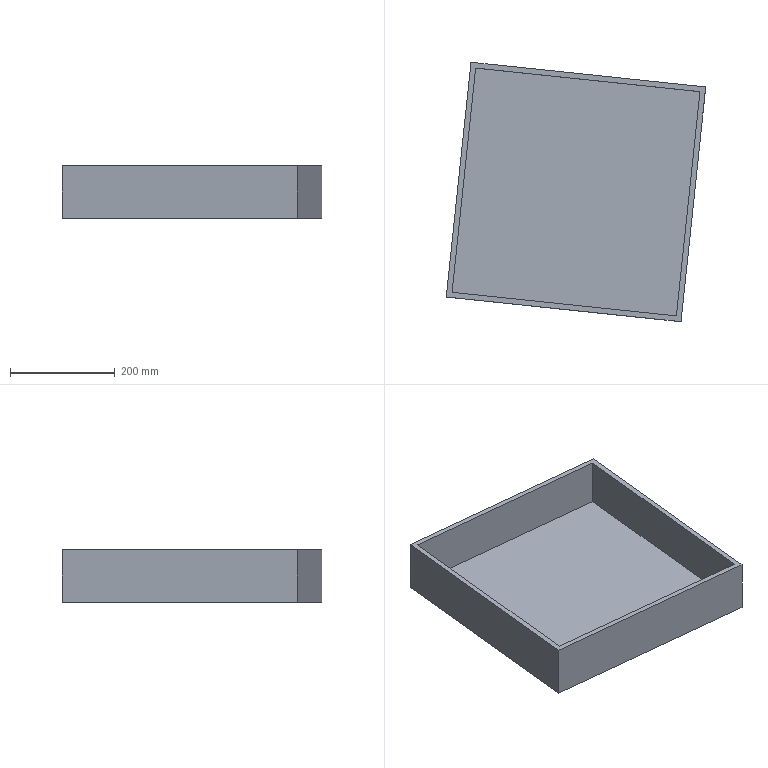Component | NX | STORAGE_BOX | 1 solid | 11 faces | box 494.57 x 494.57 x 100 mm | volume 3609000 mm3 | plane 11
STEP:
#1=CARTESIAN_POINT('',(0.,0.,0.));
#2=DIRECTION('',(0.,0.,1.));
#3=DIRECTION('',(1.,0.,0.));
#4=AXIS2_PLACEMENT_3D('',#1,#2,#3);
#5=CARTESIAN_POINT('',(1089.335,1116.284,120.));
#6=VERTEX_POINT('',#5);
#7=CARTESIAN_POINT('',(1042.297,668.75,120.));
#8=VERTEX_POINT('',#7);
#9=CARTESIAN_POINT('',(1065.816,892.517,120.));
#10=DIRECTION('',(-0.1045,-0.9945,0.));
#11=VECTOR('',#10,1.);
#12=LINE('',#9,#11);
#13=CARTESIAN_POINT('',(842.048,916.036,120.));
#14=DIRECTION('',(0.,0.,1.));
#15=DIRECTION('',(0.1045,0.9945,0.));
#16=AXIS2_PLACEMENT_3D('',#13,#14,#15);
#17=PLANE('',#16);
#18=CARTESIAN_POINT('',(-0.,-225.));
#19=DIRECTION('',(-1.,0.));
#20=VECTOR('',#19,1.);
#21=LINE('',#18,#20);
#22=(GEOMETRIC_REPRESENTATION_CONTEXT(2)PARAMETRIC_REPRESENTATION_CONTEXT()REPRESENTATION_CONTEXT('',''));
#23=DEFINITIONAL_REPRESENTATION('',(#21),#22);
#24=PCURVE('',#17,#23);
#25=CARTESIAN_POINT('',(1065.816,892.517,20.));
#26=DIRECTION('',(0.9945,-0.1045,0.));
#27=DIRECTION('',(0.,0.,-1.));
#28=AXIS2_PLACEMENT_3D('',#25,#26,#27);
#29=PLANE('',#28);
#30=CARTESIAN_POINT('',(-100.,0.));
#31=DIRECTION('',(0.,-1.));
#32=VECTOR('',#31,1.);
#33=LINE('',#30,#32);
#34=(GEOMETRIC_REPRESENTATION_CONTEXT(2)PARAMETRIC_REPRESENTATION_CONTEXT()REPRESENTATION_CONTEXT('',''));
#35=DEFINITIONAL_REPRESENTATION('',(#33),#34);
#36=PCURVE('',#29,#35);
#37=SURFACE_CURVE('',#12,(#24,#36),.PCURVE_S1.);
#38=EDGE_CURVE('',#6,#8,#37,.T.);
#39=ORIENTED_EDGE('',*,*,#38,.F.);
#40=CARTESIAN_POINT('',(641.8,1163.322,120.));
#41=VERTEX_POINT('',#40);
#42=CARTESIAN_POINT('',(865.567,1139.803,120.));
#43=DIRECTION('',(0.9945,-0.1045,0.));
#44=VECTOR('',#43,1.);
#45=LINE('',#42,#44);
#46=CARTESIAN_POINT('',(225.,-0.));
#47=DIRECTION('',(0.,-1.));
#48=VECTOR('',#47,1.);
#49=LINE('',#46,#48);
#50=(GEOMETRIC_REPRESENTATION_CONTEXT(2)PARAMETRIC_REPRESENTATION_CONTEXT()REPRESENTATION_CONTEXT('',''));
#51=DEFINITIONAL_REPRESENTATION('',(#49),#50);
#52=PCURVE('',#17,#51);
#53=CARTESIAN_POINT('',(865.567,1139.803,20.));
#54=DIRECTION('',(0.1045,0.9945,0.));
#55=DIRECTION('',(0.,0.,-1.));
#56=AXIS2_PLACEMENT_3D('',#53,#54,#55);
#57=PLANE('',#56);
#58=CARTESIAN_POINT('',(-100.,0.));
#59=DIRECTION('',(0.,-1.));
#60=VECTOR('',#59,1.);
#61=LINE('',#58,#60);
#62=(GEOMETRIC_REPRESENTATION_CONTEXT(2)PARAMETRIC_REPRESENTATION_CONTEXT()REPRESENTATION_CONTEXT('',''));
#63=DEFINITIONAL_REPRESENTATION('',(#61),#62);
#64=PCURVE('',#57,#63);
#65=SURFACE_CURVE('',#45,(#52,#64),.PCURVE_S1.);
#66=EDGE_CURVE('',#41,#6,#65,.T.);
#67=ORIENTED_EDGE('',*,*,#66,.F.);
#68=CARTESIAN_POINT('',(594.762,715.787,120.));
#69=VERTEX_POINT('',#68);
#70=CARTESIAN_POINT('',(618.281,939.555,120.));
#71=DIRECTION('',(0.1045,0.9945,0.));
#72=VECTOR('',#71,1.);
#73=LINE('',#70,#72);
#74=CARTESIAN_POINT('',(-0.,225.));
#75=DIRECTION('',(1.,0.));
#76=VECTOR('',#75,1.);
#77=LINE('',#74,#76);
#78=(GEOMETRIC_REPRESENTATION_CONTEXT(2)PARAMETRIC_REPRESENTATION_CONTEXT()REPRESENTATION_CONTEXT('',''));
#79=DEFINITIONAL_REPRESENTATION('',(#77),#78);
#80=PCURVE('',#17,#79);
#81=CARTESIAN_POINT('',(618.281,939.555,20.));
#82=DIRECTION('',(-0.9945,0.1045,0.));
#83=DIRECTION('',(0.,0.,1.));
#84=AXIS2_PLACEMENT_3D('',#81,#82,#83);
#85=PLANE('',#84);
#86=CARTESIAN_POINT('',(100.,0.));
#87=DIRECTION('',(0.,1.));
#88=VECTOR('',#87,1.);
#89=LINE('',#86,#88);
#90=(GEOMETRIC_REPRESENTATION_CONTEXT(2)PARAMETRIC_REPRESENTATION_CONTEXT()REPRESENTATION_CONTEXT('',''));
#91=DEFINITIONAL_REPRESENTATION('',(#89),#90);
#92=PCURVE('',#85,#91);
#93=SURFACE_CURVE('',#73,(#80,#92),.PCURVE_S1.);
#94=EDGE_CURVE('',#69,#41,#93,.T.);
#95=ORIENTED_EDGE('',*,*,#94,.F.);
#96=CARTESIAN_POINT('',(818.529,692.268,120.));
#97=DIRECTION('',(-0.9945,0.1045,0.));
#98=VECTOR('',#97,1.);
#99=LINE('',#96,#98);
#100=CARTESIAN_POINT('',(-225.,-0.));
#101=DIRECTION('',(0.,1.));
#102=VECTOR('',#101,1.);
#103=LINE('',#100,#102);
#104=(GEOMETRIC_REPRESENTATION_CONTEXT(2)PARAMETRIC_REPRESENTATION_CONTEXT()REPRESENTATION_CONTEXT('',''));
#105=DEFINITIONAL_REPRESENTATION('',(#103),#104);
#106=PCURVE('',#17,#105);
#107=CARTESIAN_POINT('',(818.529,692.268,20.));
#108=DIRECTION('',(-0.1045,-0.9945,0.));
#109=DIRECTION('',(0.,0.,1.));
#110=AXIS2_PLACEMENT_3D('',#107,#108,#109);
#111=PLANE('',#110);
#112=CARTESIAN_POINT('',(100.,0.));
#113=DIRECTION('',(0.,1.));
#114=VECTOR('',#113,1.);
#115=LINE('',#112,#114);
#116=(GEOMETRIC_REPRESENTATION_CONTEXT(2)PARAMETRIC_REPRESENTATION_CONTEXT()REPRESENTATION_CONTEXT('',''));
#117=DEFINITIONAL_REPRESENTATION('',(#115),#116);
#118=PCURVE('',#111,#117);
#119=SURFACE_CURVE('',#99,(#106,#118),.PCURVE_S1.);
#120=EDGE_CURVE('',#8,#69,#119,.T.);
#121=ORIENTED_EDGE('',*,*,#120,.F.);
#122=EDGE_LOOP('',(#39,#67,#95,#121));
#123=FACE_BOUND('',#122,.T.);
#124=CARTESIAN_POINT('',(650.7,1152.332,120.));
#125=VERTEX_POINT('',#124);
#126=CARTESIAN_POINT('',(1078.344,1107.384,120.));
#127=VERTEX_POINT('',#126);
#128=CARTESIAN_POINT('',(864.522,1129.858,120.));
#129=DIRECTION('',(0.9945,-0.1045,0.));
#130=VECTOR('',#129,1.);
#131=LINE('',#128,#130);
#132=CARTESIAN_POINT('',(215.,0.));
#133=DIRECTION('',(0.,-1.));
#134=VECTOR('',#133,1.);
#135=LINE('',#132,#134);
#136=(GEOMETRIC_REPRESENTATION_CONTEXT(2)PARAMETRIC_REPRESENTATION_CONTEXT()REPRESENTATION_CONTEXT('',''));
#137=DEFINITIONAL_REPRESENTATION('',(#135),#136);
#138=PCURVE('',#17,#137);
#139=CARTESIAN_POINT('',(864.522,1129.858,20.));
#140=DIRECTION('',(0.1045,0.9945,0.));
#141=DIRECTION('',(0.,0.,-1.));
#142=AXIS2_PLACEMENT_3D('',#139,#140,#141);
#143=PLANE('',#142);
#144=CARTESIAN_POINT('',(-100.,0.));
#145=DIRECTION('',(0.,-1.));
#146=VECTOR('',#145,1.);
#147=LINE('',#144,#146);
#148=(GEOMETRIC_REPRESENTATION_CONTEXT(2)PARAMETRIC_REPRESENTATION_CONTEXT()REPRESENTATION_CONTEXT('',''));
#149=DEFINITIONAL_REPRESENTATION('',(#147),#148);
#150=PCURVE('',#143,#149);
#151=SURFACE_CURVE('',#131,(#138,#150),.PCURVE_S1.);
#152=EDGE_CURVE('',#125,#127,#151,.T.);
#153=ORIENTED_EDGE('',*,*,#152,.T.);
#154=CARTESIAN_POINT('',(1033.397,679.74,120.));
#155=VERTEX_POINT('',#154);
#156=CARTESIAN_POINT('',(1055.871,893.562,120.));
#157=DIRECTION('',(-0.1045,-0.9945,0.));
#158=VECTOR('',#157,1.);
#159=LINE('',#156,#158);
#160=CARTESIAN_POINT('',(-0.,-215.));
#161=DIRECTION('',(-1.,0.));
#162=VECTOR('',#161,1.);
#163=LINE('',#160,#162);
#164=(GEOMETRIC_REPRESENTATION_CONTEXT(2)PARAMETRIC_REPRESENTATION_CONTEXT()REPRESENTATION_CONTEXT('',''));
#165=DEFINITIONAL_REPRESENTATION('',(#163),#164);
#166=PCURVE('',#17,#165);
#167=CARTESIAN_POINT('',(1055.871,893.562,20.));
#168=DIRECTION('',(0.9945,-0.1045,0.));
#169=DIRECTION('',(0.,0.,-1.));
#170=AXIS2_PLACEMENT_3D('',#167,#168,#169);
#171=PLANE('',#170);
#172=CARTESIAN_POINT('',(-100.,0.));
#173=DIRECTION('',(0.,-1.));
#174=VECTOR('',#173,1.);
#175=LINE('',#172,#174);
#176=(GEOMETRIC_REPRESENTATION_CONTEXT(2)PARAMETRIC_REPRESENTATION_CONTEXT()REPRESENTATION_CONTEXT('',''));
#177=DEFINITIONAL_REPRESENTATION('',(#175),#176);
#178=PCURVE('',#171,#177);
#179=SURFACE_CURVE('',#159,(#166,#178),.PCURVE_S1.);
#180=EDGE_CURVE('',#127,#155,#179,.T.);
#181=ORIENTED_EDGE('',*,*,#180,.T.);
#182=CARTESIAN_POINT('',(605.753,724.687,120.));
#183=VERTEX_POINT('',#182);
#184=CARTESIAN_POINT('',(819.575,702.214,120.));
#185=DIRECTION('',(-0.9945,0.1045,0.));
#186=VECTOR('',#185,1.);
#187=LINE('',#184,#186);
#188=CARTESIAN_POINT('',(-215.,0.));
#189=DIRECTION('',(0.,1.));
#190=VECTOR('',#189,1.);
#191=LINE('',#188,#190);
#192=(GEOMETRIC_REPRESENTATION_CONTEXT(2)PARAMETRIC_REPRESENTATION_CONTEXT()REPRESENTATION_CONTEXT('',''));
#193=DEFINITIONAL_REPRESENTATION('',(#191),#192);
#194=PCURVE('',#17,#193);
#195=CARTESIAN_POINT('',(819.575,702.214,20.));
#196=DIRECTION('',(-0.1045,-0.9945,0.));
#197=DIRECTION('',(0.,0.,1.));
#198=AXIS2_PLACEMENT_3D('',#195,#196,#197);
#199=PLANE('',#198);
#200=CARTESIAN_POINT('',(100.,0.));
#201=DIRECTION('',(0.,1.));
#202=VECTOR('',#201,1.);
#203=LINE('',#200,#202);
#204=(GEOMETRIC_REPRESENTATION_CONTEXT(2)PARAMETRIC_REPRESENTATION_CONTEXT()REPRESENTATION_CONTEXT('',''));
#205=DEFINITIONAL_REPRESENTATION('',(#203),#204);
#206=PCURVE('',#199,#205);
#207=SURFACE_CURVE('',#187,(#194,#206),.PCURVE_S1.);
#208=EDGE_CURVE('',#155,#183,#207,.T.);
#209=ORIENTED_EDGE('',*,*,#208,.T.);
#210=CARTESIAN_POINT('',(628.226,938.509,120.));
#211=DIRECTION('',(0.1045,0.9945,0.));
#212=VECTOR('',#211,1.);
#213=LINE('',#210,#212);
#214=CARTESIAN_POINT('',(-0.,215.));
#215=DIRECTION('',(1.,0.));
#216=VECTOR('',#215,1.);
#217=LINE('',#214,#216);
#218=(GEOMETRIC_REPRESENTATION_CONTEXT(2)PARAMETRIC_REPRESENTATION_CONTEXT()REPRESENTATION_CONTEXT('',''));
#219=DEFINITIONAL_REPRESENTATION('',(#217),#218);
#220=PCURVE('',#17,#219);
#221=CARTESIAN_POINT('',(628.226,938.509,20.));
#222=DIRECTION('',(-0.9945,0.1045,0.));
#223=DIRECTION('',(0.,0.,1.));
#224=AXIS2_PLACEMENT_3D('',#221,#222,#223);
#225=PLANE('',#224);
#226=CARTESIAN_POINT('',(100.,0.));
#227=DIRECTION('',(0.,1.));
#228=VECTOR('',#227,1.);
#229=LINE('',#226,#228);
#230=(GEOMETRIC_REPRESENTATION_CONTEXT(2)PARAMETRIC_REPRESENTATION_CONTEXT()REPRESENTATION_CONTEXT('',''));
#231=DEFINITIONAL_REPRESENTATION('',(#229),#230);
#232=PCURVE('',#225,#231);
#233=SURFACE_CURVE('',#213,(#220,#232),.PCURVE_S1.);
#234=EDGE_CURVE('',#183,#125,#233,.T.);
#235=ORIENTED_EDGE('',*,*,#234,.T.);
#236=EDGE_LOOP('',(#153,#181,#209,#235));
#237=FACE_BOUND('',#236,.T.);
#238=ADVANCED_FACE('',(#123,#237),#17,.T.);
#239=CARTESIAN_POINT('',(1089.335,1116.284,20.));
#240=VERTEX_POINT('',#239);
#241=CARTESIAN_POINT('',(1089.335,1116.284,20.));
#242=DIRECTION('',(0.,0.,1.));
#243=VECTOR('',#242,1.);
#244=LINE('',#241,#243);
#245=CARTESIAN_POINT('',(0.,225.));
#246=DIRECTION('',(-1.,0.));
#247=VECTOR('',#246,1.);
#248=LINE('',#245,#247);
#249=(GEOMETRIC_REPRESENTATION_CONTEXT(2)PARAMETRIC_REPRESENTATION_CONTEXT()REPRESENTATION_CONTEXT('',''));
#250=DEFINITIONAL_REPRESENTATION('',(#248),#249);
#251=PCURVE('',#29,#250);
#252=CARTESIAN_POINT('',(0.,-225.));
#253=DIRECTION('',(-1.,0.));
#254=VECTOR('',#253,1.);
#255=LINE('',#252,#254);
#256=(GEOMETRIC_REPRESENTATION_CONTEXT(2)PARAMETRIC_REPRESENTATION_CONTEXT()REPRESENTATION_CONTEXT('',''));
#257=DEFINITIONAL_REPRESENTATION('',(#255),#256);
#258=PCURVE('',#57,#257);
#259=SURFACE_CURVE('',#244,(#251,#258),.PCURVE_S1.);
#260=EDGE_CURVE('',#240,#6,#259,.T.);
#261=ORIENTED_EDGE('',*,*,#260,.T.);
#262=ORIENTED_EDGE('',*,*,#38,.T.);
#263=CARTESIAN_POINT('',(1042.297,668.75,20.));
#264=VERTEX_POINT('',#263);
#265=CARTESIAN_POINT('',(1042.297,668.75,20.));
#266=DIRECTION('',(0.,0.,1.));
#267=VECTOR('',#266,1.);
#268=LINE('',#265,#267);
#269=CARTESIAN_POINT('',(0.,-225.));
#270=DIRECTION('',(-1.,0.));
#271=VECTOR('',#270,1.);
#272=LINE('',#269,#271);
#273=(GEOMETRIC_REPRESENTATION_CONTEXT(2)PARAMETRIC_REPRESENTATION_CONTEXT()REPRESENTATION_CONTEXT('',''));
#274=DEFINITIONAL_REPRESENTATION('',(#272),#273);
#275=PCURVE('',#29,#274);
#276=CARTESIAN_POINT('',(0.,-225.));
#277=DIRECTION('',(1.,0.));
#278=VECTOR('',#277,1.);
#279=LINE('',#276,#278);
#280=(GEOMETRIC_REPRESENTATION_CONTEXT(2)PARAMETRIC_REPRESENTATION_CONTEXT()REPRESENTATION_CONTEXT('',''));
#281=DEFINITIONAL_REPRESENTATION('',(#279),#280);
#282=PCURVE('',#111,#281);
#283=SURFACE_CURVE('',#268,(#275,#282),.PCURVE_S1.);
#284=EDGE_CURVE('',#264,#8,#283,.T.);
#285=ORIENTED_EDGE('',*,*,#284,.F.);
#286=CARTESIAN_POINT('',(1065.816,892.517,20.));
#287=DIRECTION('',(0.1045,0.9945,0.));
#288=VECTOR('',#287,1.);
#289=LINE('',#286,#288);
#290=CARTESIAN_POINT('',(0.,0.));
#291=DIRECTION('',(0.,1.));
#292=VECTOR('',#291,1.);
#293=LINE('',#290,#292);
#294=(GEOMETRIC_REPRESENTATION_CONTEXT(2)PARAMETRIC_REPRESENTATION_CONTEXT()REPRESENTATION_CONTEXT('',''));
#295=DEFINITIONAL_REPRESENTATION('',(#293),#294);
#296=PCURVE('',#29,#295);
#297=CARTESIAN_POINT('',(842.048,916.036,20.));
#298=DIRECTION('',(0.,0.,-1.));
#299=DIRECTION('',(-0.1045,-0.9945,0.));
#300=AXIS2_PLACEMENT_3D('',#297,#298,#299);
#301=PLANE('',#300);
#302=CARTESIAN_POINT('',(0.,-225.));
#303=DIRECTION('',(-1.,0.));
#304=VECTOR('',#303,1.);
#305=LINE('',#302,#304);
#306=(GEOMETRIC_REPRESENTATION_CONTEXT(2)PARAMETRIC_REPRESENTATION_CONTEXT()REPRESENTATION_CONTEXT('',''));
#307=DEFINITIONAL_REPRESENTATION('',(#305),#306);
#308=PCURVE('',#301,#307);
#309=SURFACE_CURVE('',#289,(#296,#308),.PCURVE_S1.);
#310=EDGE_CURVE('',#264,#240,#309,.T.);
#311=ORIENTED_EDGE('',*,*,#310,.T.);
#312=EDGE_LOOP('',(#261,#262,#285,#311));
#313=FACE_BOUND('',#312,.T.);
#314=ADVANCED_FACE('',(#313),#29,.T.);
#315=ORIENTED_EDGE('',*,*,#284,.T.);
#316=ORIENTED_EDGE('',*,*,#120,.T.);
#317=CARTESIAN_POINT('',(594.762,715.787,20.));
#318=VERTEX_POINT('',#317);
#319=CARTESIAN_POINT('',(594.762,715.787,20.));
#320=DIRECTION('',(0.,0.,1.));
#321=VECTOR('',#320,1.);
#322=LINE('',#319,#321);
#323=CARTESIAN_POINT('',(0.,225.));
#324=DIRECTION('',(1.,0.));
#325=VECTOR('',#324,1.);
#326=LINE('',#323,#325);
#327=(GEOMETRIC_REPRESENTATION_CONTEXT(2)PARAMETRIC_REPRESENTATION_CONTEXT()REPRESENTATION_CONTEXT('',''));
#328=DEFINITIONAL_REPRESENTATION('',(#326),#327);
#329=PCURVE('',#111,#328);
#330=CARTESIAN_POINT('',(0.,-225.));
#331=DIRECTION('',(1.,0.));
#332=VECTOR('',#331,1.);
#333=LINE('',#330,#332);
#334=(GEOMETRIC_REPRESENTATION_CONTEXT(2)PARAMETRIC_REPRESENTATION_CONTEXT()REPRESENTATION_CONTEXT('',''));
#335=DEFINITIONAL_REPRESENTATION('',(#333),#334);
#336=PCURVE('',#85,#335);
#337=SURFACE_CURVE('',#322,(#329,#336),.PCURVE_S1.);
#338=EDGE_CURVE('',#318,#69,#337,.T.);
#339=ORIENTED_EDGE('',*,*,#338,.F.);
#340=CARTESIAN_POINT('',(818.529,692.268,20.));
#341=DIRECTION('',(0.9945,-0.1045,0.));
#342=VECTOR('',#341,1.);
#343=LINE('',#340,#342);
#344=CARTESIAN_POINT('',(0.,0.));
#345=DIRECTION('',(0.,-1.));
#346=VECTOR('',#345,1.);
#347=LINE('',#344,#346);
#348=(GEOMETRIC_REPRESENTATION_CONTEXT(2)PARAMETRIC_REPRESENTATION_CONTEXT()REPRESENTATION_CONTEXT('',''));
#349=DEFINITIONAL_REPRESENTATION('',(#347),#348);
#350=PCURVE('',#111,#349);
#351=CARTESIAN_POINT('',(225.,-0.));
#352=DIRECTION('',(0.,-1.));
#353=VECTOR('',#352,1.);
#354=LINE('',#351,#353);
#355=(GEOMETRIC_REPRESENTATION_CONTEXT(2)PARAMETRIC_REPRESENTATION_CONTEXT()REPRESENTATION_CONTEXT('',''));
#356=DEFINITIONAL_REPRESENTATION('',(#354),#355);
#357=PCURVE('',#301,#356);
#358=SURFACE_CURVE('',#343,(#350,#357),.PCURVE_S1.);
#359=EDGE_CURVE('',#318,#264,#358,.T.);
#360=ORIENTED_EDGE('',*,*,#359,.T.);
#361=EDGE_LOOP('',(#315,#316,#339,#360));
#362=FACE_BOUND('',#361,.T.);
#363=ADVANCED_FACE('',(#362),#111,.T.);
#364=ORIENTED_EDGE('',*,*,#338,.T.);
#365=ORIENTED_EDGE('',*,*,#94,.T.);
#366=CARTESIAN_POINT('',(641.8,1163.322,20.));
#367=VERTEX_POINT('',#366);
#368=CARTESIAN_POINT('',(641.8,1163.322,20.));
#369=DIRECTION('',(0.,0.,1.));
#370=VECTOR('',#369,1.);
#371=LINE('',#368,#370);
#372=CARTESIAN_POINT('',(0.,225.));
#373=DIRECTION('',(1.,0.));
#374=VECTOR('',#373,1.);
#375=LINE('',#372,#374);
#376=(GEOMETRIC_REPRESENTATION_CONTEXT(2)PARAMETRIC_REPRESENTATION_CONTEXT()REPRESENTATION_CONTEXT('',''));
#377=DEFINITIONAL_REPRESENTATION('',(#375),#376);
#378=PCURVE('',#85,#377);
#379=CARTESIAN_POINT('',(0.,225.));
#380=DIRECTION('',(-1.,0.));
#381=VECTOR('',#380,1.);
#382=LINE('',#379,#381);
#383=(GEOMETRIC_REPRESENTATION_CONTEXT(2)PARAMETRIC_REPRESENTATION_CONTEXT()REPRESENTATION_CONTEXT('',''));
#384=DEFINITIONAL_REPRESENTATION('',(#382),#383);
#385=PCURVE('',#57,#384);
#386=SURFACE_CURVE('',#371,(#378,#385),.PCURVE_S1.);
#387=EDGE_CURVE('',#367,#41,#386,.T.);
#388=ORIENTED_EDGE('',*,*,#387,.F.);
#389=CARTESIAN_POINT('',(618.281,939.555,20.));
#390=DIRECTION('',(-0.1045,-0.9945,0.));
#391=VECTOR('',#390,1.);
#392=LINE('',#389,#391);
#393=CARTESIAN_POINT('',(0.,0.));
#394=DIRECTION('',(0.,-1.));
#395=VECTOR('',#394,1.);
#396=LINE('',#393,#395);
#397=(GEOMETRIC_REPRESENTATION_CONTEXT(2)PARAMETRIC_REPRESENTATION_CONTEXT()REPRESENTATION_CONTEXT('',''));
#398=DEFINITIONAL_REPRESENTATION('',(#396),#397);
#399=PCURVE('',#85,#398);
#400=CARTESIAN_POINT('',(0.,225.));
#401=DIRECTION('',(1.,0.));
#402=VECTOR('',#401,1.);
#403=LINE('',#400,#402);
#404=(GEOMETRIC_REPRESENTATION_CONTEXT(2)PARAMETRIC_REPRESENTATION_CONTEXT()REPRESENTATION_CONTEXT('',''));
#405=DEFINITIONAL_REPRESENTATION('',(#403),#404);
#406=PCURVE('',#301,#405);
#407=SURFACE_CURVE('',#392,(#399,#406),.PCURVE_S1.);
#408=EDGE_CURVE('',#367,#318,#407,.T.);
#409=ORIENTED_EDGE('',*,*,#408,.T.);
#410=EDGE_LOOP('',(#364,#365,#388,#409));
#411=FACE_BOUND('',#410,.T.);
#412=ADVANCED_FACE('',(#411),#85,.T.);
#413=CARTESIAN_POINT('',(865.567,1139.803,20.));
#414=DIRECTION('',(-0.9945,0.1045,0.));
#415=VECTOR('',#414,1.);
#416=LINE('',#413,#415);
#417=CARTESIAN_POINT('',(-225.,-0.));
#418=DIRECTION('',(0.,1.));
#419=VECTOR('',#418,1.);
#420=LINE('',#417,#419);
#421=(GEOMETRIC_REPRESENTATION_CONTEXT(2)PARAMETRIC_REPRESENTATION_CONTEXT()REPRESENTATION_CONTEXT('',''));
#422=DEFINITIONAL_REPRESENTATION('',(#420),#421);
#423=PCURVE('',#301,#422);
#424=CARTESIAN_POINT('',(0.,0.));
#425=DIRECTION('',(0.,1.));
#426=VECTOR('',#425,1.);
#427=LINE('',#424,#426);
#428=(GEOMETRIC_REPRESENTATION_CONTEXT(2)PARAMETRIC_REPRESENTATION_CONTEXT()REPRESENTATION_CONTEXT('',''));
#429=DEFINITIONAL_REPRESENTATION('',(#427),#428);
#430=PCURVE('',#57,#429);
#431=SURFACE_CURVE('',#416,(#423,#430),.PCURVE_S1.);
#432=EDGE_CURVE('',#240,#367,#431,.T.);
#433=ORIENTED_EDGE('',*,*,#432,.F.);
#434=ORIENTED_EDGE('',*,*,#310,.F.);
#435=ORIENTED_EDGE('',*,*,#359,.F.);
#436=ORIENTED_EDGE('',*,*,#408,.F.);
#437=EDGE_LOOP('',(#433,#434,#435,#436));
#438=FACE_BOUND('',#437,.T.);
#439=ADVANCED_FACE('',(#438),#301,.T.);
#440=ORIENTED_EDGE('',*,*,#432,.T.);
#441=ORIENTED_EDGE('',*,*,#387,.T.);
#442=ORIENTED_EDGE('',*,*,#66,.T.);
#443=ORIENTED_EDGE('',*,*,#260,.F.);
#444=EDGE_LOOP('',(#440,#441,#442,#443));
#445=FACE_BOUND('',#444,.T.);
#446=ADVANCED_FACE('',(#445),#57,.T.);
#447=CARTESIAN_POINT('',(1078.344,1107.384,30.));
#448=VERTEX_POINT('',#447);
#449=CARTESIAN_POINT('',(1078.344,1107.384,20.));
#450=DIRECTION('',(0.,0.,1.));
#451=VECTOR('',#450,1.);
#452=LINE('',#449,#451);
#453=CARTESIAN_POINT('',(0.,215.));
#454=DIRECTION('',(-1.,0.));
#455=VECTOR('',#454,1.);
#456=LINE('',#453,#455);
#457=(GEOMETRIC_REPRESENTATION_CONTEXT(2)PARAMETRIC_REPRESENTATION_CONTEXT()REPRESENTATION_CONTEXT('',''));
#458=DEFINITIONAL_REPRESENTATION('',(#456),#457);
#459=PCURVE('',#171,#458);
#460=CARTESIAN_POINT('',(0.,-215.));
#461=DIRECTION('',(-1.,0.));
#462=VECTOR('',#461,1.);
#463=LINE('',#460,#462);
#464=(GEOMETRIC_REPRESENTATION_CONTEXT(2)PARAMETRIC_REPRESENTATION_CONTEXT()REPRESENTATION_CONTEXT('',''));
#465=DEFINITIONAL_REPRESENTATION('',(#463),#464);
#466=PCURVE('',#143,#465);
#467=SURFACE_CURVE('',#452,(#459,#466),.PCURVE_S1.);
#468=EDGE_CURVE('',#448,#127,#467,.T.);
#469=ORIENTED_EDGE('',*,*,#468,.F.);
#470=CARTESIAN_POINT('',(1033.397,679.74,30.));
#471=VERTEX_POINT('',#470);
#472=CARTESIAN_POINT('',(1055.871,893.562,30.));
#473=DIRECTION('',(0.1045,0.9945,0.));
#474=VECTOR('',#473,1.);
#475=LINE('',#472,#474);
#476=CARTESIAN_POINT('',(-10.,0.));
#477=DIRECTION('',(0.,1.));
#478=VECTOR('',#477,1.);
#479=LINE('',#476,#478);
#480=(GEOMETRIC_REPRESENTATION_CONTEXT(2)PARAMETRIC_REPRESENTATION_CONTEXT()REPRESENTATION_CONTEXT('',''));
#481=DEFINITIONAL_REPRESENTATION('',(#479),#480);
#482=PCURVE('',#171,#481);
#483=CARTESIAN_POINT('',(842.048,916.036,30.));
#484=DIRECTION('',(0.,0.,-1.));
#485=DIRECTION('',(-0.1045,-0.9945,0.));
#486=AXIS2_PLACEMENT_3D('',#483,#484,#485);
#487=PLANE('',#486);
#488=CARTESIAN_POINT('',(0.,-215.));
#489=DIRECTION('',(-1.,0.));
#490=VECTOR('',#489,1.);
#491=LINE('',#488,#490);
#492=(GEOMETRIC_REPRESENTATION_CONTEXT(2)PARAMETRIC_REPRESENTATION_CONTEXT()REPRESENTATION_CONTEXT('',''));
#493=DEFINITIONAL_REPRESENTATION('',(#491),#492);
#494=PCURVE('',#487,#493);
#495=SURFACE_CURVE('',#475,(#482,#494),.PCURVE_S1.);
#496=EDGE_CURVE('',#471,#448,#495,.T.);
#497=ORIENTED_EDGE('',*,*,#496,.F.);
#498=CARTESIAN_POINT('',(1033.397,679.74,20.));
#499=DIRECTION('',(0.,0.,1.));
#500=VECTOR('',#499,1.);
#501=LINE('',#498,#500);
#502=CARTESIAN_POINT('',(0.,-215.));
#503=DIRECTION('',(-1.,0.));
#504=VECTOR('',#503,1.);
#505=LINE('',#502,#504);
#506=(GEOMETRIC_REPRESENTATION_CONTEXT(2)PARAMETRIC_REPRESENTATION_CONTEXT()REPRESENTATION_CONTEXT('',''));
#507=DEFINITIONAL_REPRESENTATION('',(#505),#506);
#508=PCURVE('',#171,#507);
#509=CARTESIAN_POINT('',(0.,-215.));
#510=DIRECTION('',(1.,0.));
#511=VECTOR('',#510,1.);
#512=LINE('',#509,#511);
#513=(GEOMETRIC_REPRESENTATION_CONTEXT(2)PARAMETRIC_REPRESENTATION_CONTEXT()REPRESENTATION_CONTEXT('',''));
#514=DEFINITIONAL_REPRESENTATION('',(#512),#513);
#515=PCURVE('',#199,#514);
#516=SURFACE_CURVE('',#501,(#508,#515),.PCURVE_S1.);
#517=EDGE_CURVE('',#471,#155,#516,.T.);
#518=ORIENTED_EDGE('',*,*,#517,.T.);
#519=ORIENTED_EDGE('',*,*,#180,.F.);
#520=EDGE_LOOP('',(#469,#497,#518,#519));
#521=FACE_BOUND('',#520,.T.);
#522=ADVANCED_FACE('',(#521),#171,.F.);
#523=ORIENTED_EDGE('',*,*,#517,.F.);
#524=CARTESIAN_POINT('',(605.753,724.687,30.));
#525=VERTEX_POINT('',#524);
#526=CARTESIAN_POINT('',(819.575,702.214,30.));
#527=DIRECTION('',(0.9945,-0.1045,0.));
#528=VECTOR('',#527,1.);
#529=LINE('',#526,#528);
#530=CARTESIAN_POINT('',(10.,0.));
#531=DIRECTION('',(0.,-1.));
#532=VECTOR('',#531,1.);
#533=LINE('',#530,#532);
#534=(GEOMETRIC_REPRESENTATION_CONTEXT(2)PARAMETRIC_REPRESENTATION_CONTEXT()REPRESENTATION_CONTEXT('',''));
#535=DEFINITIONAL_REPRESENTATION('',(#533),#534);
#536=PCURVE('',#199,#535);
#537=CARTESIAN_POINT('',(215.,0.));
#538=DIRECTION('',(0.,-1.));
#539=VECTOR('',#538,1.);
#540=LINE('',#537,#539);
#541=(GEOMETRIC_REPRESENTATION_CONTEXT(2)PARAMETRIC_REPRESENTATION_CONTEXT()REPRESENTATION_CONTEXT('',''));
#542=DEFINITIONAL_REPRESENTATION('',(#540),#541);
#543=PCURVE('',#487,#542);
#544=SURFACE_CURVE('',#529,(#536,#543),.PCURVE_S1.);
#545=EDGE_CURVE('',#525,#471,#544,.T.);
#546=ORIENTED_EDGE('',*,*,#545,.F.);
#547=CARTESIAN_POINT('',(605.753,724.687,20.));
#548=DIRECTION('',(0.,0.,1.));
#549=VECTOR('',#548,1.);
#550=LINE('',#547,#549);
#551=CARTESIAN_POINT('',(0.,215.));
#552=DIRECTION('',(1.,0.));
#553=VECTOR('',#552,1.);
#554=LINE('',#551,#553);
#555=(GEOMETRIC_REPRESENTATION_CONTEXT(2)PARAMETRIC_REPRESENTATION_CONTEXT()REPRESENTATION_CONTEXT('',''));
#556=DEFINITIONAL_REPRESENTATION('',(#554),#555);
#557=PCURVE('',#199,#556);
#558=CARTESIAN_POINT('',(0.,-215.));
#559=DIRECTION('',(1.,0.));
#560=VECTOR('',#559,1.);
#561=LINE('',#558,#560);
#562=(GEOMETRIC_REPRESENTATION_CONTEXT(2)PARAMETRIC_REPRESENTATION_CONTEXT()REPRESENTATION_CONTEXT('',''));
#563=DEFINITIONAL_REPRESENTATION('',(#561),#562);
#564=PCURVE('',#225,#563);
#565=SURFACE_CURVE('',#550,(#557,#564),.PCURVE_S1.);
#566=EDGE_CURVE('',#525,#183,#565,.T.);
#567=ORIENTED_EDGE('',*,*,#566,.T.);
#568=ORIENTED_EDGE('',*,*,#208,.F.);
#569=EDGE_LOOP('',(#523,#546,#567,#568));
#570=FACE_BOUND('',#569,.T.);
#571=ADVANCED_FACE('',(#570),#199,.F.);
#572=ORIENTED_EDGE('',*,*,#566,.F.);
#573=CARTESIAN_POINT('',(650.7,1152.332,30.));
#574=VERTEX_POINT('',#573);
#575=CARTESIAN_POINT('',(628.226,938.509,30.));
#576=DIRECTION('',(-0.1045,-0.9945,0.));
#577=VECTOR('',#576,1.);
#578=LINE('',#575,#577);
#579=CARTESIAN_POINT('',(10.,0.));
#580=DIRECTION('',(0.,-1.));
#581=VECTOR('',#580,1.);
#582=LINE('',#579,#581);
#583=(GEOMETRIC_REPRESENTATION_CONTEXT(2)PARAMETRIC_REPRESENTATION_CONTEXT()REPRESENTATION_CONTEXT('',''));
#584=DEFINITIONAL_REPRESENTATION('',(#582),#583);
#585=PCURVE('',#225,#584);
#586=CARTESIAN_POINT('',(0.,215.));
#587=DIRECTION('',(1.,0.));
#588=VECTOR('',#587,1.);
#589=LINE('',#586,#588);
#590=(GEOMETRIC_REPRESENTATION_CONTEXT(2)PARAMETRIC_REPRESENTATION_CONTEXT()REPRESENTATION_CONTEXT('',''));
#591=DEFINITIONAL_REPRESENTATION('',(#589),#590);
#592=PCURVE('',#487,#591);
#593=SURFACE_CURVE('',#578,(#585,#592),.PCURVE_S1.);
#594=EDGE_CURVE('',#574,#525,#593,.T.);
#595=ORIENTED_EDGE('',*,*,#594,.F.);
#596=CARTESIAN_POINT('',(650.7,1152.332,20.));
#597=DIRECTION('',(0.,0.,1.));
#598=VECTOR('',#597,1.);
#599=LINE('',#596,#598);
#600=CARTESIAN_POINT('',(0.,215.));
#601=DIRECTION('',(1.,0.));
#602=VECTOR('',#601,1.);
#603=LINE('',#600,#602);
#604=(GEOMETRIC_REPRESENTATION_CONTEXT(2)PARAMETRIC_REPRESENTATION_CONTEXT()REPRESENTATION_CONTEXT('',''));
#605=DEFINITIONAL_REPRESENTATION('',(#603),#604);
#606=PCURVE('',#225,#605);
#607=CARTESIAN_POINT('',(0.,215.));
#608=DIRECTION('',(-1.,0.));
#609=VECTOR('',#608,1.);
#610=LINE('',#607,#609);
#611=(GEOMETRIC_REPRESENTATION_CONTEXT(2)PARAMETRIC_REPRESENTATION_CONTEXT()REPRESENTATION_CONTEXT('',''));
#612=DEFINITIONAL_REPRESENTATION('',(#610),#611);
#613=PCURVE('',#143,#612);
#614=SURFACE_CURVE('',#599,(#606,#613),.PCURVE_S1.);
#615=EDGE_CURVE('',#574,#125,#614,.T.);
#616=ORIENTED_EDGE('',*,*,#615,.T.);
#617=ORIENTED_EDGE('',*,*,#234,.F.);
#618=EDGE_LOOP('',(#572,#595,#616,#617));
#619=FACE_BOUND('',#618,.T.);
#620=ADVANCED_FACE('',(#619),#225,.F.);
#621=CARTESIAN_POINT('',(864.522,1129.858,30.));
#622=DIRECTION('',(-0.9945,0.1045,0.));
#623=VECTOR('',#622,1.);
#624=LINE('',#621,#623);
#625=CARTESIAN_POINT('',(-215.,0.));
#626=DIRECTION('',(0.,1.));
#627=VECTOR('',#626,1.);
#628=LINE('',#625,#627);
#629=(GEOMETRIC_REPRESENTATION_CONTEXT(2)PARAMETRIC_REPRESENTATION_CONTEXT()REPRESENTATION_CONTEXT('',''));
#630=DEFINITIONAL_REPRESENTATION('',(#628),#629);
#631=PCURVE('',#487,#630);
#632=CARTESIAN_POINT('',(-10.,0.));
#633=DIRECTION('',(0.,1.));
#634=VECTOR('',#633,1.);
#635=LINE('',#632,#634);
#636=(GEOMETRIC_REPRESENTATION_CONTEXT(2)PARAMETRIC_REPRESENTATION_CONTEXT()REPRESENTATION_CONTEXT('',''));
#637=DEFINITIONAL_REPRESENTATION('',(#635),#636);
#638=PCURVE('',#143,#637);
#639=SURFACE_CURVE('',#624,(#631,#638),.PCURVE_S1.);
#640=EDGE_CURVE('',#448,#574,#639,.T.);
#641=ORIENTED_EDGE('',*,*,#640,.T.);
#642=ORIENTED_EDGE('',*,*,#594,.T.);
#643=ORIENTED_EDGE('',*,*,#545,.T.);
#644=ORIENTED_EDGE('',*,*,#496,.T.);
#645=EDGE_LOOP('',(#641,#642,#643,#644));
#646=FACE_BOUND('',#645,.T.);
#647=ADVANCED_FACE('',(#646),#487,.F.);
#648=ORIENTED_EDGE('',*,*,#640,.F.);
#649=ORIENTED_EDGE('',*,*,#468,.T.);
#650=ORIENTED_EDGE('',*,*,#152,.F.);
#651=ORIENTED_EDGE('',*,*,#615,.F.);
#652=EDGE_LOOP('',(#648,#649,#650,#651));
#653=FACE_BOUND('',#652,.T.);
#654=ADVANCED_FACE('',(#653),#143,.F.);
#655=CLOSED_SHELL('',(#238,#314,#363,#412,#439,#446,#522,#571,#620,#647,#654));
#656=MANIFOLD_SOLID_BREP('',#655);
#657=(LENGTH_UNIT()NAMED_UNIT(*)SI_UNIT(.MILLI.,.METRE.));
#658=UNCERTAINTY_MEASURE_WITH_UNIT(LENGTH_MEASURE(0.0000001),#657,'','');
#659=(NAMED_UNIT(*)PLANE_ANGLE_UNIT()SI_UNIT($,.RADIAN.));
#660=(NAMED_UNIT(*)SI_UNIT($,.STERADIAN.)SOLID_ANGLE_UNIT());
#661=(GEOMETRIC_REPRESENTATION_CONTEXT(3)GLOBAL_UNCERTAINTY_ASSIGNED_CONTEXT((#658))GLOBAL_UNIT_ASSIGNED_CONTEXT((#657,#659,#660))REPRESENTATION_CONTEXT('',''));
#662=ADVANCED_BREP_SHAPE_REPRESENTATION('',(#4,#656),#661);